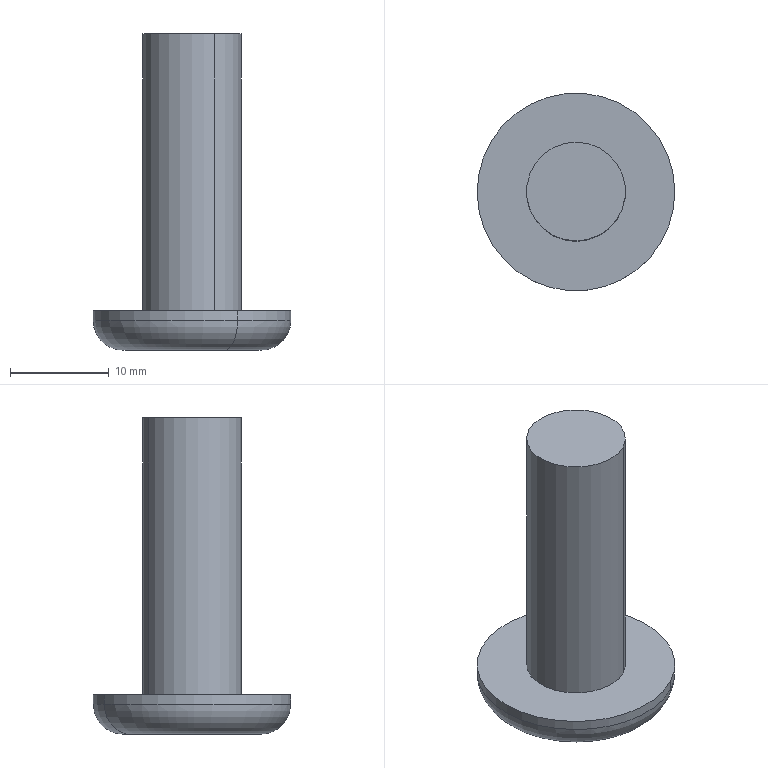Component | SolidWorks | FixedPin24mm-2 | 1 solid | 9 faces | box 20 x 20 x 32 mm | volume 3343 mm3 | cylinder 4 | plane 3 | torus 2 | commonest cylinder face diameters 20 x2 10 x2
build123d program:
from build123d import *

# Parameters (mm, degrees)
SKETCH1_R           = 5
BOSS_EXTRUDE1_DEPTH = 28
SKETCH2_R           = 10
BOSS_EXTRUDE2_DEPTH = 4
FILLET1_R           = 3


with BuildPart() as part:
    # Sketch1 → Boss-Extrude1 (new body)
    with BuildSketch(Plane.XY):
        Circle(SKETCH1_R)
    extrude(amount=BOSS_EXTRUDE1_DEPTH)

    # Sketch2 → Boss-Extrude2 (add)
    with BuildSketch(Plane.XY.offset(28)):
        Circle(SKETCH2_R)
    extrude(amount=BOSS_EXTRUDE2_DEPTH)

    # Fillet1
    fillet1_edges = [part.edges().sort_by_distance(p)[0] for p in [
        (-10, 0, 32),
    ]]
    fillet(fillet1_edges, radius=FILLET1_R)


solid = part.part

# Placed as in the assembly
solid = solid.moved(Location((21.07, -11.003, 136.846), (180, 0, 0)))
STEP:
#1=COLOUR_RGB('',0.7922,0.8196,0.9333);
#2=FILL_AREA_STYLE_COLOUR('',#1);
#3=FILL_AREA_STYLE('',(#2));
#4=SURFACE_STYLE_FILL_AREA(#3);
#5=SURFACE_SIDE_STYLE('',(#4));
#6=SURFACE_STYLE_USAGE(.BOTH.,#5);
#7=PRESENTATION_STYLE_ASSIGNMENT((#6));
#8=CARTESIAN_POINT('',(0.6475,-0.08406,4.246));
#9=VERTEX_POINT('',#8);
#10=CARTESIAN_POINT('',(1.012,-0.7823,4.246));
#11=VERTEX_POINT('',#10);
#12=CARTESIAN_POINT('',(0.8295,-0.4332,4.246));
#13=DIRECTION('',(0.,0.,1.));
#14=DIRECTION('',(0.4622,-0.8868,0.));
#15=AXIS2_PLACEMENT_3D('',#12,#13,#14);
#16=CIRCLE('',#15,0.3937);
#17=EDGE_CURVE('',#9,#11,#16,.T.);
#18=ORIENTED_EDGE('',*,*,#17,.F.);
#19=CARTESIAN_POINT('',(0.7021,-0.1888,4.128));
#20=VERTEX_POINT('',#19);
#21=CARTESIAN_POINT('',(0.7021,-0.1888,4.246));
#22=DIRECTION('',(-0.8868,-0.4622,0.));
#23=DIRECTION('',(0.4622,-0.8868,0.));
#24=AXIS2_PLACEMENT_3D('',#21,#22,#23);
#25=CIRCLE('',#24,0.1181);
#26=EDGE_CURVE('',#9,#20,#25,.T.);
#27=ORIENTED_EDGE('',*,*,#26,.T.);
#28=CARTESIAN_POINT('',(0.9569,-0.6776,4.128));
#29=VERTEX_POINT('',#28);
#30=CARTESIAN_POINT('',(0.8295,-0.4332,4.128));
#31=DIRECTION('',(0.,0.,-1.));
#32=DIRECTION('',(0.4622,-0.8868,0.));
#33=AXIS2_PLACEMENT_3D('',#30,#31,#32);
#34=CIRCLE('',#33,0.2756);
#35=EDGE_CURVE('',#29,#20,#34,.T.);
#36=ORIENTED_EDGE('',*,*,#35,.F.);
#37=CARTESIAN_POINT('',(0.9569,-0.6776,4.246));
#38=DIRECTION('',(0.8868,0.4622,0.));
#39=DIRECTION('',(-0.4622,0.8868,0.));
#40=AXIS2_PLACEMENT_3D('',#37,#38,#39);
#41=CIRCLE('',#40,0.1181);
#42=EDGE_CURVE('',#11,#29,#41,.T.);
#43=ORIENTED_EDGE('',*,*,#42,.F.);
#44=EDGE_LOOP('',(#18,#27,#36,#43));
#45=FACE_OUTER_BOUND('',#44,.T.);
#46=CARTESIAN_POINT('',(0.8295,-0.4332,4.246));
#47=DIRECTION('',(0.,0.,-1.));
#48=DIRECTION('',(0.4622,-0.8868,0.));
#49=AXIS2_PLACEMENT_3D('',#46,#47,#48);
#50=TOROIDAL_SURFACE('',#49,0.2756,0.1181);
#51=ADVANCED_FACE('',(#45),#50,.T.);
#52=ORIENTED_EDGE('',*,*,#17,.T.);
#53=CARTESIAN_POINT('',(1.012,-0.7823,4.285));
#54=VERTEX_POINT('',#53);
#55=CARTESIAN_POINT('',(1.012,-0.7823,4.128));
#56=DIRECTION('',(0.,0.,1.));
#57=VECTOR('',#56,39.37);
#58=LINE('',#55,#57);
#59=EDGE_CURVE('',#11,#54,#58,.T.);
#60=ORIENTED_EDGE('',*,*,#59,.T.);
#61=CARTESIAN_POINT('',(0.6475,-0.08406,4.285));
#62=VERTEX_POINT('',#61);
#63=CARTESIAN_POINT('',(0.8295,-0.4332,4.285));
#64=DIRECTION('',(0.,0.,-1.));
#65=DIRECTION('',(0.4622,-0.8868,0.));
#66=AXIS2_PLACEMENT_3D('',#63,#64,#65);
#67=CIRCLE('',#66,0.3937);
#68=EDGE_CURVE('',#54,#62,#67,.T.);
#69=ORIENTED_EDGE('',*,*,#68,.T.);
#70=CARTESIAN_POINT('',(0.6475,-0.08406,4.128));
#71=DIRECTION('',(0.,0.,1.));
#72=VECTOR('',#71,39.37);
#73=LINE('',#70,#72);
#74=EDGE_CURVE('',#9,#62,#73,.T.);
#75=ORIENTED_EDGE('',*,*,#74,.F.);
#76=EDGE_LOOP('',(#52,#60,#69,#75));
#77=FACE_OUTER_BOUND('',#76,.T.);
#78=CARTESIAN_POINT('',(0.8295,-0.4332,4.128));
#79=DIRECTION('',(0.,0.,1.));
#80=DIRECTION('',(-0.4622,0.8868,0.));
#81=AXIS2_PLACEMENT_3D('',#78,#79,#80);
#82=CYLINDRICAL_SURFACE('',#81,0.3937);
#83=ADVANCED_FACE('',(#77),#82,.T.);
#84=CARTESIAN_POINT('',(0.9205,-0.6077,4.285));
#85=VERTEX_POINT('',#84);
#86=CARTESIAN_POINT('',(0.7385,-0.2586,4.285));
#87=VERTEX_POINT('',#86);
#88=CARTESIAN_POINT('',(0.8295,-0.4332,4.285));
#89=DIRECTION('',(0.,0.,-1.));
#90=DIRECTION('',(0.4622,-0.8868,0.));
#91=AXIS2_PLACEMENT_3D('',#88,#89,#90);
#92=CIRCLE('',#91,0.1969);
#93=EDGE_CURVE('',#85,#87,#92,.T.);
#94=ORIENTED_EDGE('',*,*,#93,.F.);
#95=CARTESIAN_POINT('',(0.9205,-0.6077,5.388));
#96=VERTEX_POINT('',#95);
#97=CARTESIAN_POINT('',(0.9205,-0.6077,4.285));
#98=DIRECTION('',(0.,0.,1.));
#99=VECTOR('',#98,39.37);
#100=LINE('',#97,#99);
#101=EDGE_CURVE('',#85,#96,#100,.T.);
#102=ORIENTED_EDGE('',*,*,#101,.T.);
#103=CARTESIAN_POINT('',(0.7385,-0.2586,5.388));
#104=VERTEX_POINT('',#103);
#105=CARTESIAN_POINT('',(0.8295,-0.4332,5.388));
#106=DIRECTION('',(0.,0.,-1.));
#107=DIRECTION('',(0.4622,-0.8868,0.));
#108=AXIS2_PLACEMENT_3D('',#105,#106,#107);
#109=CIRCLE('',#108,0.1969);
#110=EDGE_CURVE('',#96,#104,#109,.T.);
#111=ORIENTED_EDGE('',*,*,#110,.T.);
#112=CARTESIAN_POINT('',(0.7385,-0.2586,4.285));
#113=DIRECTION('',(0.,0.,1.));
#114=VECTOR('',#113,39.37);
#115=LINE('',#112,#114);
#116=EDGE_CURVE('',#87,#104,#115,.T.);
#117=ORIENTED_EDGE('',*,*,#116,.F.);
#118=EDGE_LOOP('',(#94,#102,#111,#117));
#119=FACE_OUTER_BOUND('',#118,.T.);
#120=CARTESIAN_POINT('',(0.8295,-0.4332,4.285));
#121=DIRECTION('',(0.,0.,1.));
#122=DIRECTION('',(-0.4622,0.8868,0.));
#123=AXIS2_PLACEMENT_3D('',#120,#121,#122);
#124=CYLINDRICAL_SURFACE('',#123,0.1969);
#125=ADVANCED_FACE('',(#119),#124,.T.);
#126=ORIENTED_EDGE('',*,*,#101,.F.);
#127=CARTESIAN_POINT('',(0.8295,-0.4332,4.285));
#128=DIRECTION('',(0.,0.,-1.));
#129=DIRECTION('',(0.4622,-0.8868,0.));
#130=AXIS2_PLACEMENT_3D('',#127,#128,#129);
#131=CIRCLE('',#130,0.1969);
#132=EDGE_CURVE('',#87,#85,#131,.T.);
#133=ORIENTED_EDGE('',*,*,#132,.F.);
#134=ORIENTED_EDGE('',*,*,#116,.T.);
#135=CARTESIAN_POINT('',(0.8295,-0.4332,5.388));
#136=DIRECTION('',(0.,0.,-1.));
#137=DIRECTION('',(0.4622,-0.8868,0.));
#138=AXIS2_PLACEMENT_3D('',#135,#136,#137);
#139=CIRCLE('',#138,0.1969);
#140=EDGE_CURVE('',#104,#96,#139,.T.);
#141=ORIENTED_EDGE('',*,*,#140,.T.);
#142=EDGE_LOOP('',(#126,#133,#134,#141));
#143=FACE_OUTER_BOUND('',#142,.T.);
#144=CARTESIAN_POINT('',(0.8295,-0.4332,4.285));
#145=DIRECTION('',(0.,0.,1.));
#146=DIRECTION('',(-0.4622,0.8868,0.));
#147=AXIS2_PLACEMENT_3D('',#144,#145,#146);
#148=CYLINDRICAL_SURFACE('',#147,0.1969);
#149=ADVANCED_FACE('',(#143),#148,.T.);
#150=ORIENTED_EDGE('',*,*,#140,.F.);
#151=ORIENTED_EDGE('',*,*,#110,.F.);
#152=EDGE_LOOP('',(#150,#151));
#153=FACE_OUTER_BOUND('',#152,.T.);
#154=CARTESIAN_POINT('',(0.8295,-0.4332,5.388));
#155=DIRECTION('',(0.,0.,-1.));
#156=DIRECTION('',(0.4622,-0.8868,0.));
#157=AXIS2_PLACEMENT_3D('',#154,#155,#156);
#158=PLANE('',#157);
#159=ADVANCED_FACE('',(#153),#158,.F.);
#160=ORIENTED_EDGE('',*,*,#59,.F.);
#161=CARTESIAN_POINT('',(0.8295,-0.4332,4.246));
#162=DIRECTION('',(0.,0.,1.));
#163=DIRECTION('',(0.4622,-0.8868,0.));
#164=AXIS2_PLACEMENT_3D('',#161,#162,#163);
#165=CIRCLE('',#164,0.3937);
#166=EDGE_CURVE('',#11,#9,#165,.T.);
#167=ORIENTED_EDGE('',*,*,#166,.T.);
#168=ORIENTED_EDGE('',*,*,#74,.T.);
#169=CARTESIAN_POINT('',(0.8295,-0.4332,4.285));
#170=DIRECTION('',(0.,0.,-1.));
#171=DIRECTION('',(0.4622,-0.8868,0.));
#172=AXIS2_PLACEMENT_3D('',#169,#170,#171);
#173=CIRCLE('',#172,0.3937);
#174=EDGE_CURVE('',#62,#54,#173,.T.);
#175=ORIENTED_EDGE('',*,*,#174,.T.);
#176=EDGE_LOOP('',(#160,#167,#168,#175));
#177=FACE_OUTER_BOUND('',#176,.T.);
#178=CARTESIAN_POINT('',(0.8295,-0.4332,4.128));
#179=DIRECTION('',(0.,0.,1.));
#180=DIRECTION('',(-0.4622,0.8868,0.));
#181=AXIS2_PLACEMENT_3D('',#178,#179,#180);
#182=CYLINDRICAL_SURFACE('',#181,0.3937);
#183=ADVANCED_FACE('',(#177),#182,.T.);
#184=ORIENTED_EDGE('',*,*,#35,.T.);
#185=CARTESIAN_POINT('',(0.8295,-0.4332,4.128));
#186=DIRECTION('',(0.,0.,-1.));
#187=DIRECTION('',(0.4622,-0.8868,0.));
#188=AXIS2_PLACEMENT_3D('',#185,#186,#187);
#189=CIRCLE('',#188,0.2756);
#190=EDGE_CURVE('',#20,#29,#189,.T.);
#191=ORIENTED_EDGE('',*,*,#190,.T.);
#192=EDGE_LOOP('',(#184,#191));
#193=FACE_OUTER_BOUND('',#192,.T.);
#194=CARTESIAN_POINT('',(0.8295,-0.4332,4.128));
#195=DIRECTION('',(0.,0.,-1.));
#196=DIRECTION('',(0.4622,-0.8868,0.));
#197=AXIS2_PLACEMENT_3D('',#194,#195,#196);
#198=PLANE('',#197);
#199=ADVANCED_FACE('',(#193),#198,.T.);
#200=ORIENTED_EDGE('',*,*,#132,.T.);
#201=ORIENTED_EDGE('',*,*,#93,.T.);
#202=EDGE_LOOP('',(#200,#201));
#203=FACE_BOUND('',#202,.T.);
#204=ORIENTED_EDGE('',*,*,#174,.F.);
#205=ORIENTED_EDGE('',*,*,#68,.F.);
#206=EDGE_LOOP('',(#204,#205));
#207=FACE_OUTER_BOUND('',#206,.T.);
#208=CARTESIAN_POINT('',(0.8295,-0.4332,4.285));
#209=DIRECTION('',(0.,0.,-1.));
#210=DIRECTION('',(0.4622,-0.8868,0.));
#211=AXIS2_PLACEMENT_3D('',#208,#209,#210);
#212=PLANE('',#211);
#213=ADVANCED_FACE('',(#203,#207),#212,.F.);
#214=ORIENTED_EDGE('',*,*,#26,.F.);
#215=ORIENTED_EDGE('',*,*,#166,.F.);
#216=ORIENTED_EDGE('',*,*,#42,.T.);
#217=ORIENTED_EDGE('',*,*,#190,.F.);
#218=EDGE_LOOP('',(#214,#215,#216,#217));
#219=FACE_OUTER_BOUND('',#218,.T.);
#220=CARTESIAN_POINT('',(0.8295,-0.4332,4.246));
#221=DIRECTION('',(0.,0.,-1.));
#222=DIRECTION('',(0.4622,-0.8868,0.));
#223=AXIS2_PLACEMENT_3D('',#220,#221,#222);
#224=TOROIDAL_SURFACE('',#223,0.2756,0.1181);
#225=ADVANCED_FACE('',(#219),#224,.T.);
#226=CLOSED_SHELL('',(#51,#83,#125,#149,#159,#183,#199,#213,#225));
#227=MANIFOLD_SOLID_BREP('',#226);
#228=STYLED_ITEM('',(#7),#227);
#229=(LENGTH_UNIT()NAMED_UNIT(*)SI_UNIT($,.METRE.));
#230=LENGTH_MEASURE_WITH_UNIT(LENGTH_MEASURE(0.0254),#229);
#231=DIMENSIONAL_EXPONENTS(1.,0.,0.,0.,0.,0.,0.);
#232=(CONVERSION_BASED_UNIT('',#230)LENGTH_UNIT()NAMED_UNIT(#231));
#233=UNCERTAINTY_MEASURE_WITH_UNIT(LENGTH_MEASURE(0.00001),#232,'','');
#234=(NAMED_UNIT(*)PLANE_ANGLE_UNIT()SI_UNIT($,.RADIAN.));
#235=(NAMED_UNIT(*)SI_UNIT($,.STERADIAN.)SOLID_ANGLE_UNIT());
#236=(GEOMETRIC_REPRESENTATION_CONTEXT(3)GLOBAL_UNCERTAINTY_ASSIGNED_CONTEXT((#233))GLOBAL_UNIT_ASSIGNED_CONTEXT((#232,#234,#235))REPRESENTATION_CONTEXT('',''));
#237=MECHANICAL_DESIGN_GEOMETRIC_PRESENTATION_REPRESENTATION('',(#228),#236);
#238=CARTESIAN_POINT('',(0.,0.,0.));
#239=DIRECTION('',(0.,0.,1.));
#240=DIRECTION('',(1.,0.,0.));
#241=AXIS2_PLACEMENT_3D('',#238,#239,#240);
#242=(LENGTH_UNIT()NAMED_UNIT(*)SI_UNIT($,.METRE.));
#243=LENGTH_MEASURE_WITH_UNIT(LENGTH_MEASURE(0.0254),#242);
#244=DIMENSIONAL_EXPONENTS(1.,0.,0.,0.,0.,0.,0.);
#245=(CONVERSION_BASED_UNIT('',#243)LENGTH_UNIT()NAMED_UNIT(#244));
#246=UNCERTAINTY_MEASURE_WITH_UNIT(LENGTH_MEASURE(0.00001),#245,'','');
#247=(NAMED_UNIT(*)PLANE_ANGLE_UNIT()SI_UNIT($,.RADIAN.));
#248=(NAMED_UNIT(*)SI_UNIT($,.STERADIAN.)SOLID_ANGLE_UNIT());
#249=(GEOMETRIC_REPRESENTATION_CONTEXT(3)GLOBAL_UNCERTAINTY_ASSIGNED_CONTEXT((#246))GLOBAL_UNIT_ASSIGNED_CONTEXT((#245,#247,#248))REPRESENTATION_CONTEXT('',''));
#250=ADVANCED_BREP_SHAPE_REPRESENTATION('',(#227,#241),#249);
#251=PRESENTATION_LAYER_ASSIGNMENT('','',(#228));